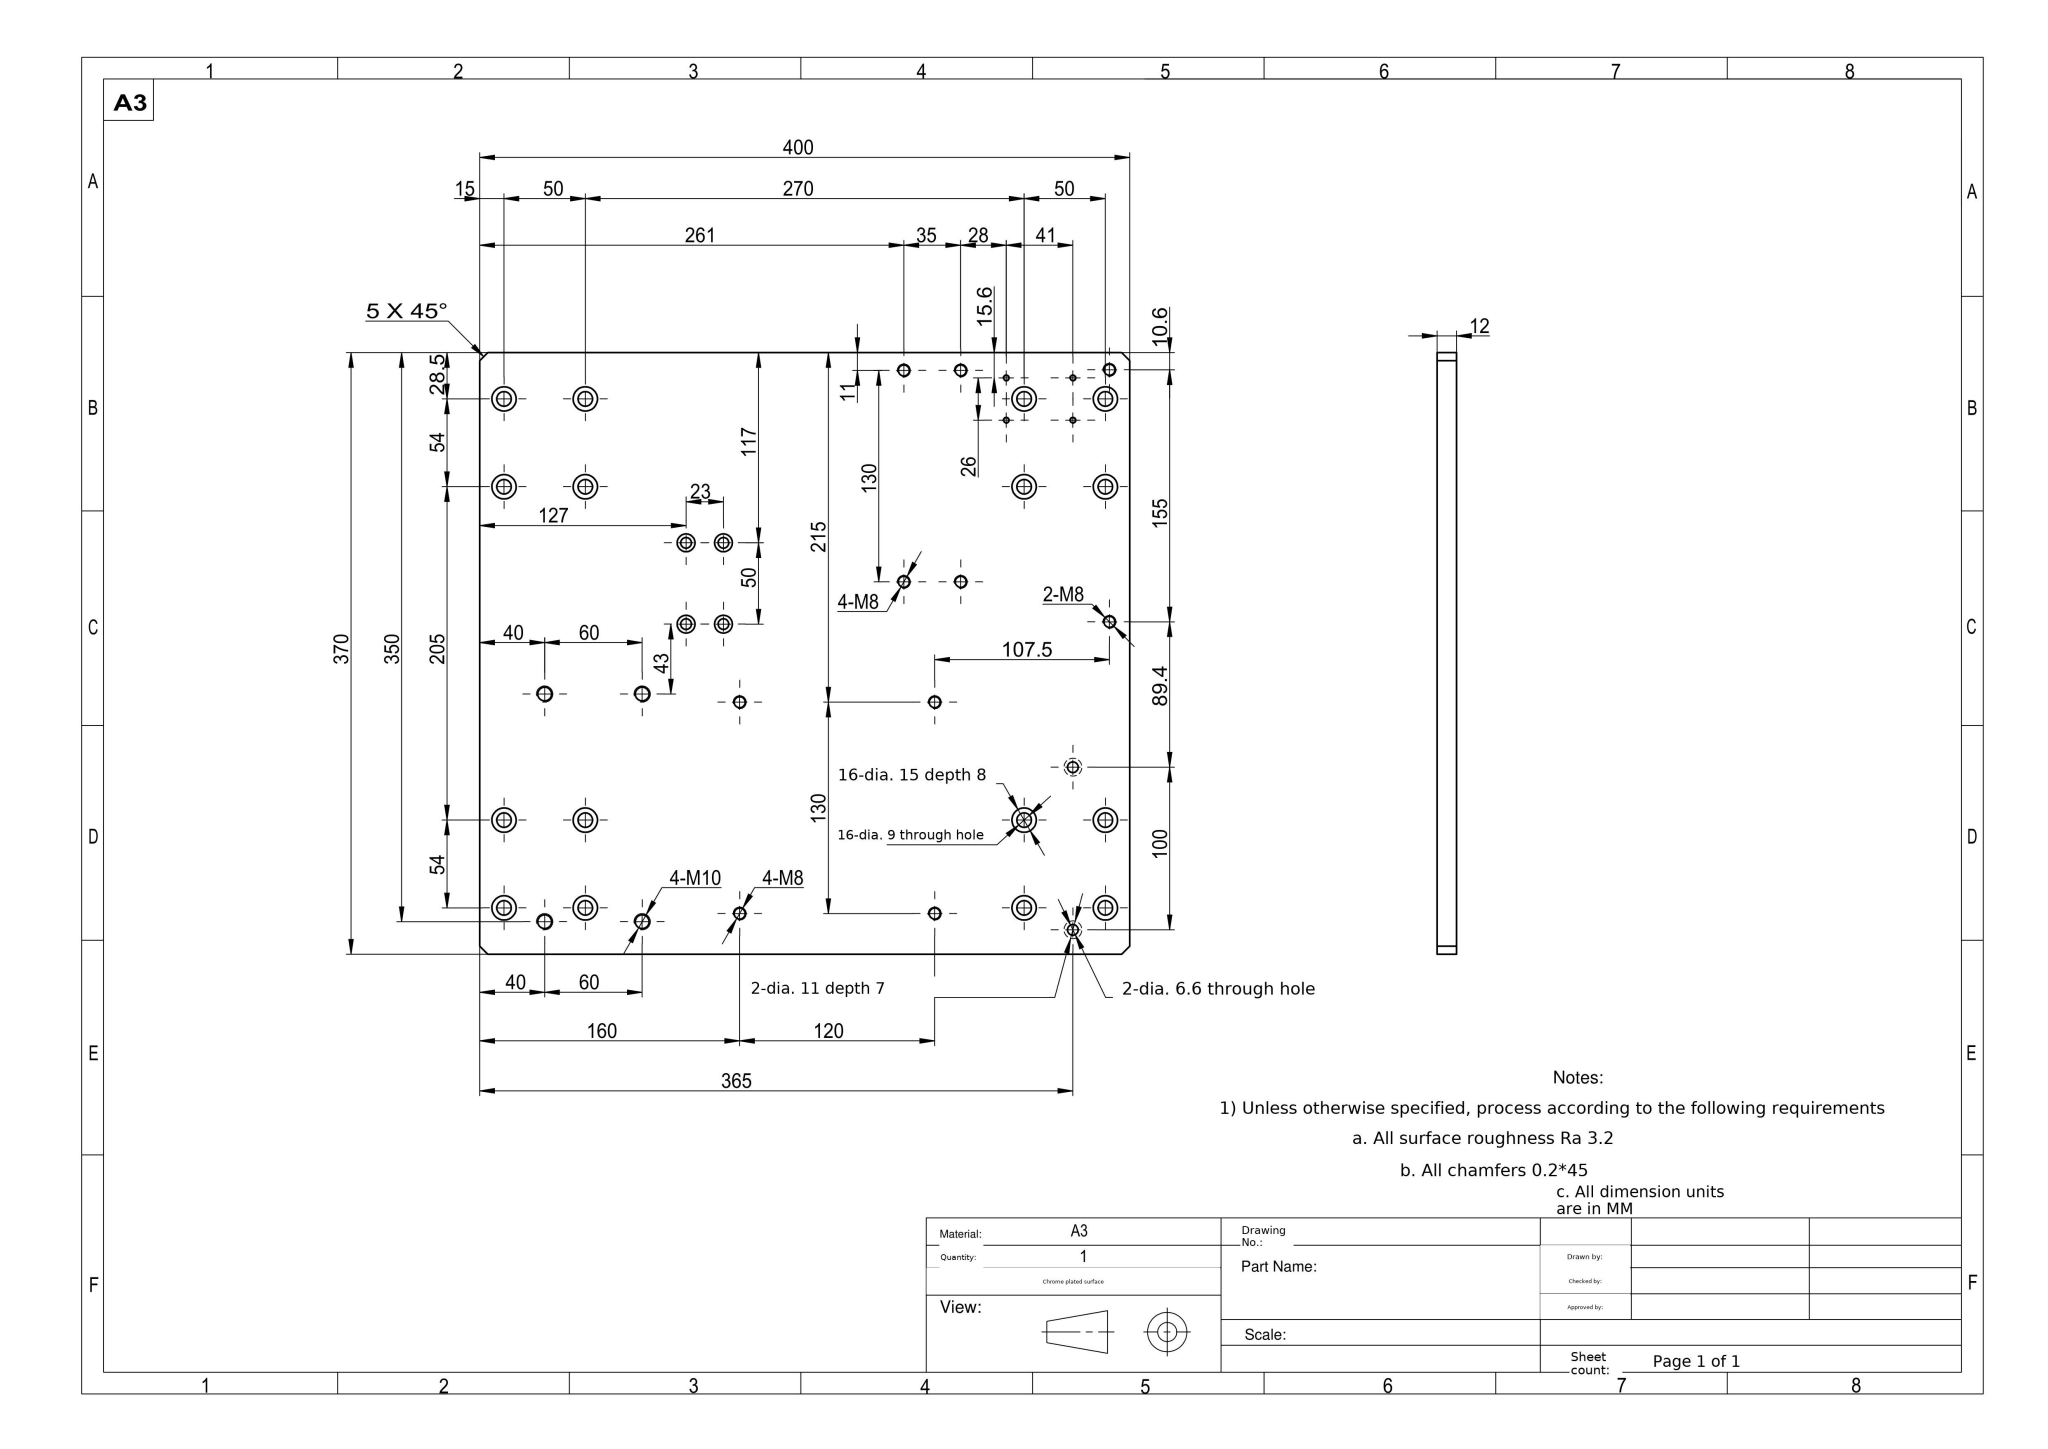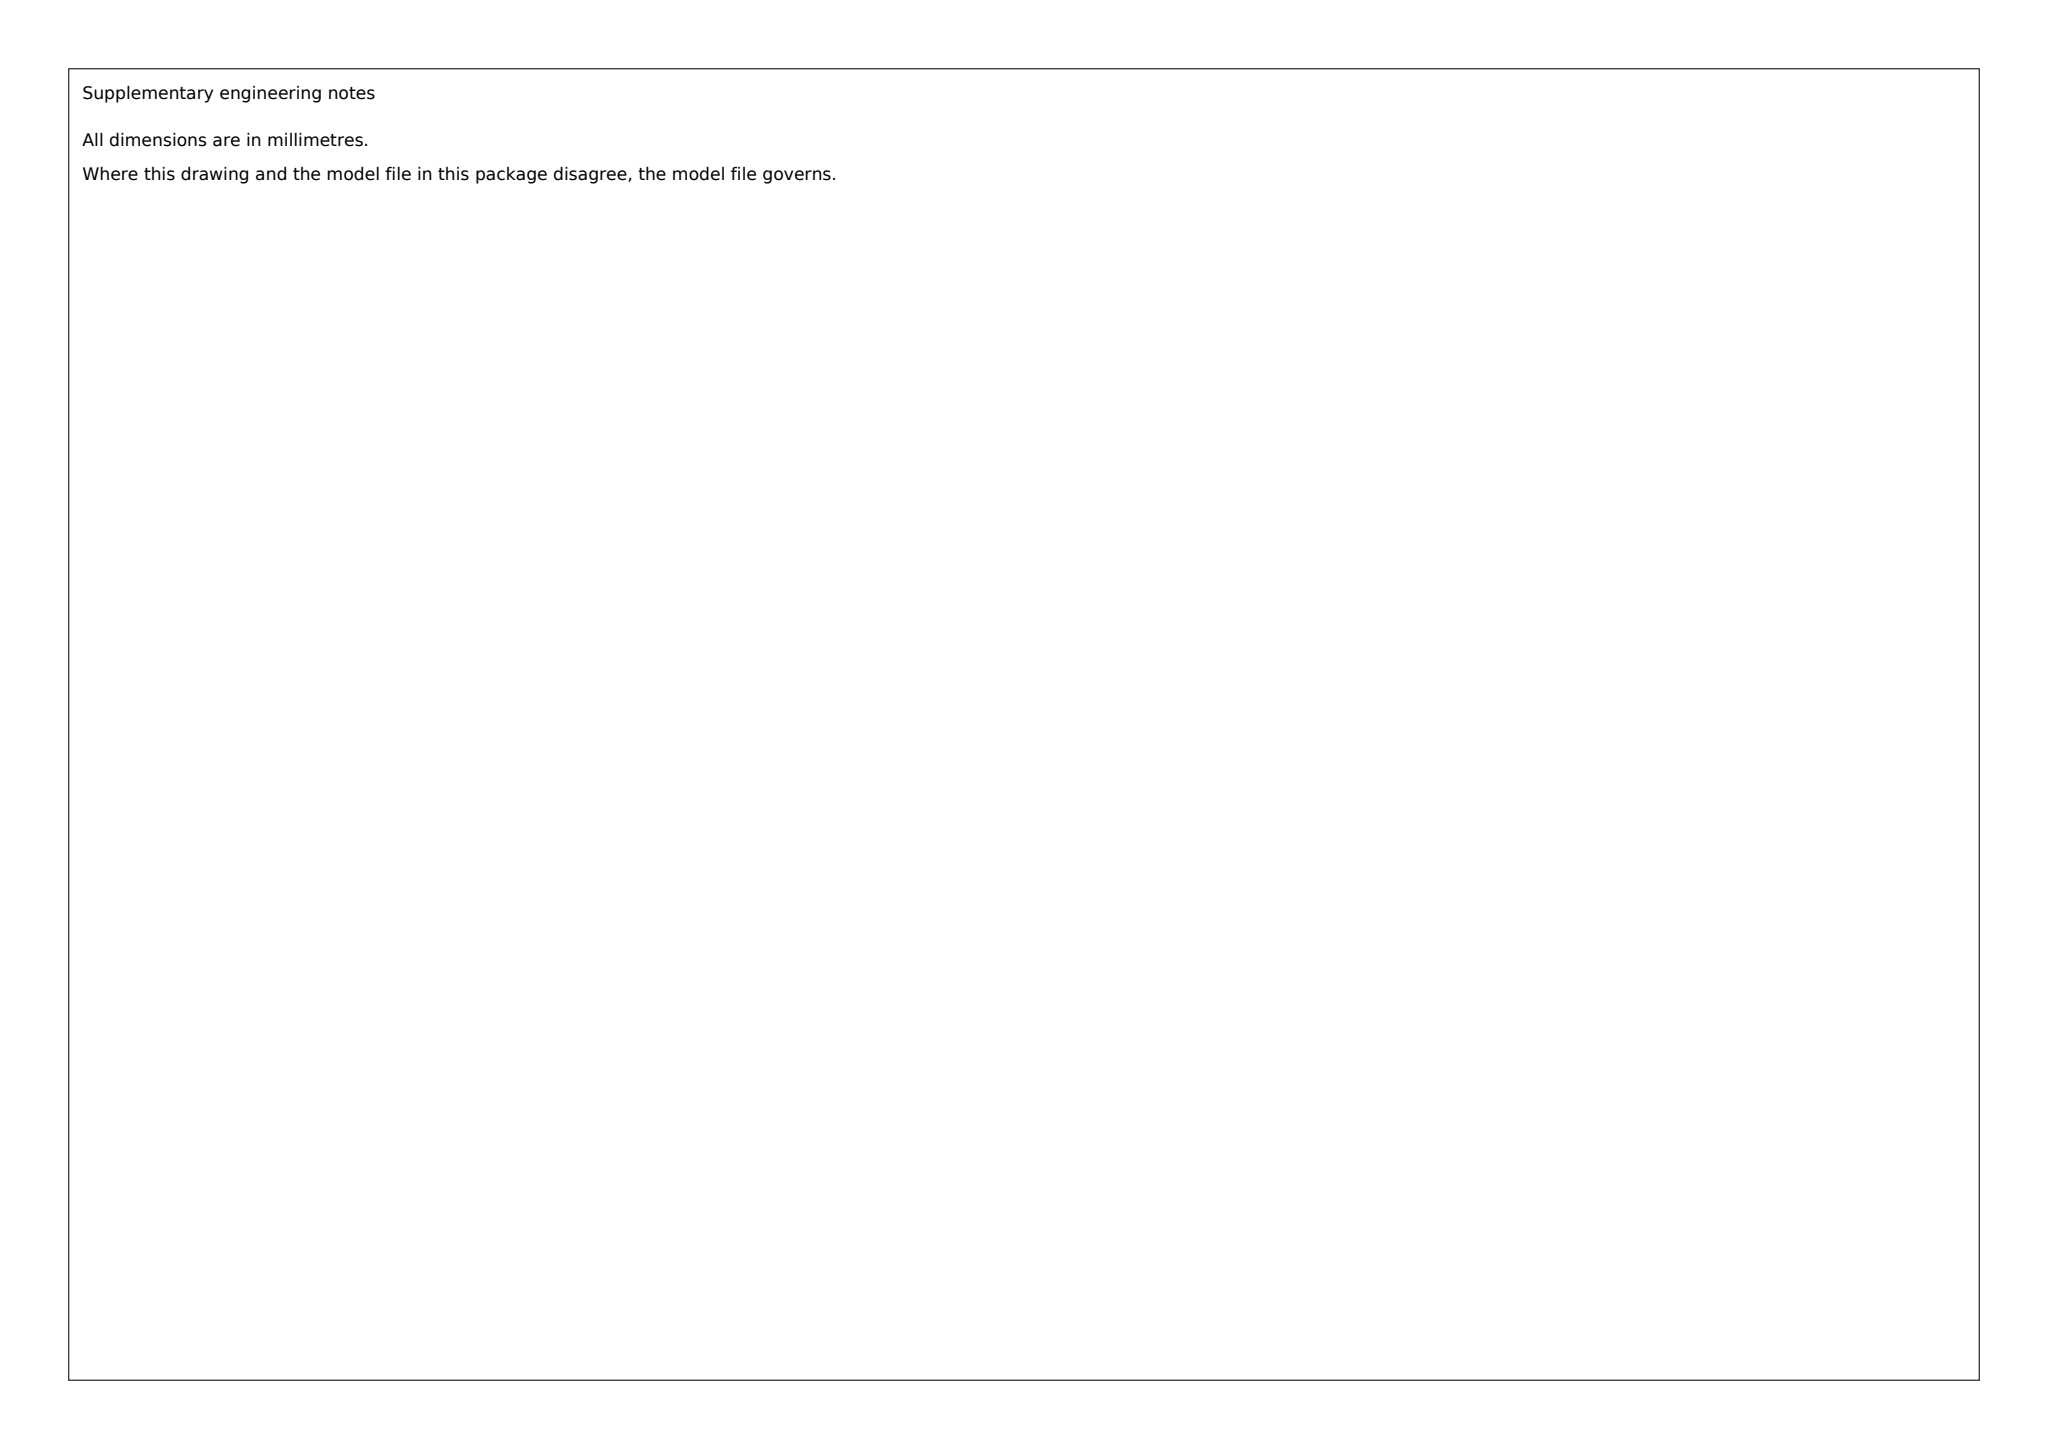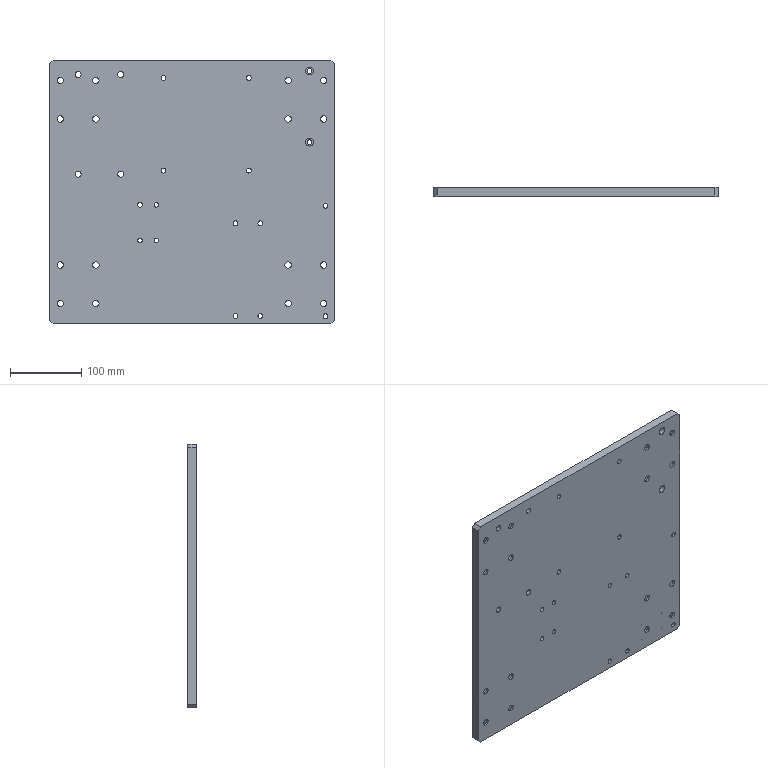Part | SolidWorks | mm | material A3 | 1 solid | 164 faces | box 400 x 12 x 370 mm | volume 1734516 mm3 | cylinder 124 | plane 32 | cone 8 | commonest cylinder face diameters 15 x32 9 x32 6.8 x20 11 x12 6.6 x12 8.5 x8 3.3 x8
build123d program:
from build123d import *

# Parameters (mm, degrees)
SKETCH1_W                                         = 400
SKETCH1_H                                         = 370
BOSS_EXTRUDE1_DEPTH                               = 6
HOLE_SIZE_ACCORDING_TO_HEXAGON_SOCKET_D           = 9
HOLE_SIZE_ACCORDING_TO_HEXAGON_SOCKET_DEPTH       = 22.25
HOLE_SIZE_ACCORDING_TO_HEXAGON_SOCKET_CBORE_D     = 15
HOLE_SIZE_ACCORDING_TO_HEXAGON_SOCKET_CBORE_DEPTH = 9
HOLE_SIZE_ACCORDING_TO_HEXAGON_SOCKET_TIP         = 2.704
HOLE_SIZE_ACCORDING_TO_HEXAGON_SO_2_D             = 6.6
HOLE_SIZE_ACCORDING_TO_HEXAGON_SO_2_DEPTH         = 15
HOLE_SIZE_ACCORDING_TO_HEXAGON_SO_2_CBORE_D       = 11
HOLE_SIZE_ACCORDING_TO_HEXAGON_SO_2_CBORE_DEPTH   = 6.8
HOLE_SIZE_ACCORDING_TO_HEXAGON_SO_2_TIP           = 1.983
M4_TAPPED_HOLE1_D                                 = 3.3
M4_TAPPED_HOLE1_DEPTH                             = 10.1
M4_TAPPED_HOLE1_TIP                               = 0.9914
M8_TAPPED_HOLE1_D                                 = 6.8
M8_TAPPED_HOLE1_DEPTH                             = 22.25
M8_TAPPED_HOLE1_TIP                               = 2.043
M8_TAPPED_HOLE2_D                                 = 6.8
M8_TAPPED_HOLE2_DEPTH                             = 19.75
M8_TAPPED_HOLE2_TIP                               = 2.043
M8_TAPPED_HOLE3_D                                 = 6.8
M8_TAPPED_HOLE3_DEPTH                             = 22.25
M8_TAPPED_HOLE3_TIP                               = 2.043
HOLE_SIZE_ACCORDING_TO_HEXAGON_SO_3_D             = 6.6
HOLE_SIZE_ACCORDING_TO_HEXAGON_SO_3_DEPTH         = 17
HOLE_SIZE_ACCORDING_TO_HEXAGON_SO_3_CBORE_D       = 11
HOLE_SIZE_ACCORDING_TO_HEXAGON_SO_3_CBORE_DEPTH   = 6.8
HOLE_SIZE_ACCORDING_TO_HEXAGON_SO_3_TIP           = 1.983
M10_TAPPED_HOLE2_D                                = 8.5
M10_TAPPED_HOLE2_DEPTH                            = 27.5
M10_TAPPED_HOLE2_TIP                              = 2.554
CHAMFER1_SIZE                                     = 5


with BuildPart() as part:
    # Sketch1 → Boss-Extrude1 (new, symmetric)
    with BuildSketch(Plane(origin=(0, 0, 0), x_dir=(1, 0, 0), z_dir=(0, 1, 0))):
        Rectangle(SKETCH1_W, SKETCH1_H)
    extrude(amount=BOSS_EXTRUDE1_DEPTH, both=True)

    # Hole Size _ according to_ Hexagon Socket
    with Locations(Plane(origin=(0, 6, 0), x_dir=(1, 0, 0), z_dir=(0, 1, 0))):
        with Locations((-185, -102.5), (-185, -156.5), (-135, -102.5), (-135, -156.5), (-135, 156.5), (-135, 102.5), (-185, 156.5), (-185, 102.5), (185, 102.5), (185, 156.5), (135, 102.5), (135, 156.5), (135, -156.5), (135, -102.5), (185, -156.5), (185, -102.5)):
            CounterBoreHole(HOLE_SIZE_ACCORDING_TO_HEXAGON_SOCKET_D / 2, HOLE_SIZE_ACCORDING_TO_HEXAGON_SOCKET_CBORE_D / 2, HOLE_SIZE_ACCORDING_TO_HEXAGON_SOCKET_CBORE_DEPTH, depth=HOLE_SIZE_ACCORDING_TO_HEXAGON_SOCKET_DEPTH)
            with Locations((0, 0, -(HOLE_SIZE_ACCORDING_TO_HEXAGON_SOCKET_DEPTH + HOLE_SIZE_ACCORDING_TO_HEXAGON_SOCKET_TIP / 2))):  # 118° drill point
                Cone(0, HOLE_SIZE_ACCORDING_TO_HEXAGON_SOCKET_D / 2, HOLE_SIZE_ACCORDING_TO_HEXAGON_SOCKET_TIP, mode=Mode.SUBTRACT)

    # Hole Size _ according to_ Hexagon So 2
    with Locations(Plane(origin=(0, -6, 0), x_dir=(-1, 0, 0), z_dir=(0, -1, 0))):
        with Locations((-165, -170), (-165, -70)):
            CounterBoreHole(HOLE_SIZE_ACCORDING_TO_HEXAGON_SO_2_D / 2, HOLE_SIZE_ACCORDING_TO_HEXAGON_SO_2_CBORE_D / 2, HOLE_SIZE_ACCORDING_TO_HEXAGON_SO_2_CBORE_DEPTH, depth=HOLE_SIZE_ACCORDING_TO_HEXAGON_SO_2_DEPTH)
            with Locations((0, 0, -(HOLE_SIZE_ACCORDING_TO_HEXAGON_SO_2_DEPTH + HOLE_SIZE_ACCORDING_TO_HEXAGON_SO_2_TIP / 2))):  # 118° drill point
                Cone(0, HOLE_SIZE_ACCORDING_TO_HEXAGON_SO_2_D / 2, HOLE_SIZE_ACCORDING_TO_HEXAGON_SO_2_TIP, mode=Mode.SUBTRACT)

    # M4 Tapped Hole1
    with Locations(Plane(origin=(0, 6, 0), x_dir=(1, 0, 0), z_dir=(0, 1, 0))):
        with Locations((124, 169.4), (124, 143.4), (165, 143.4), (165, 169.4)):
            Hole(M4_TAPPED_HOLE1_D / 2, depth=M4_TAPPED_HOLE1_DEPTH)
            with Locations((0, 0, -(M4_TAPPED_HOLE1_DEPTH + M4_TAPPED_HOLE1_TIP / 2))):  # 118° drill point
                Cone(0, M4_TAPPED_HOLE1_D / 2, M4_TAPPED_HOLE1_TIP, mode=Mode.SUBTRACT)

    # M8 Tapped Hole1
    with Locations(Plane(origin=(0, 6, 0), x_dir=(1, 0, 0), z_dir=(0, 1, 0))):
        with Locations((187.5, 19.4), (187.5, 174.4)):
            Hole(M8_TAPPED_HOLE1_D / 2, depth=M8_TAPPED_HOLE1_DEPTH)
            with Locations((0, 0, -(M8_TAPPED_HOLE1_DEPTH + M8_TAPPED_HOLE1_TIP / 2))):  # 118° drill point
                Cone(0, M8_TAPPED_HOLE1_D / 2, M8_TAPPED_HOLE1_TIP, mode=Mode.SUBTRACT)

    # M8 Tapped Hole2
    with Locations(Plane(origin=(0, 6, 0), x_dir=(1, 0, 0), z_dir=(0, 1, 0))):
        with Locations((61, 44), (61, 174), (96, 174), (96, 44)):
            Hole(M8_TAPPED_HOLE2_D / 2, depth=M8_TAPPED_HOLE2_DEPTH)
            with Locations((0, 0, -(M8_TAPPED_HOLE2_DEPTH + M8_TAPPED_HOLE2_TIP / 2))):  # 118° drill point
                Cone(0, M8_TAPPED_HOLE2_D / 2, M8_TAPPED_HOLE2_TIP, mode=Mode.SUBTRACT)

    # M8 Tapped Hole3
    with Locations(Plane(origin=(0, 6, 0), x_dir=(1, 0, 0), z_dir=(0, 1, 0))):
        with Locations((-40, -160), (80, -160), (80, -30), (-40, -30)):
            Hole(M8_TAPPED_HOLE3_D / 2, depth=M8_TAPPED_HOLE3_DEPTH)
            with Locations((0, 0, -(M8_TAPPED_HOLE3_DEPTH + M8_TAPPED_HOLE3_TIP / 2))):  # 118° drill point
                Cone(0, M8_TAPPED_HOLE3_D / 2, M8_TAPPED_HOLE3_TIP, mode=Mode.SUBTRACT)

    # Hole Size _ according to_ Hexagon So 3
    with Locations(Plane(origin=(0, 6, 0), x_dir=(1, 0, 0), z_dir=(0, 1, 0))):
        with Locations((-73, 68), (-50, 68), (-73, 18), (-50, 18)):
            CounterBoreHole(HOLE_SIZE_ACCORDING_TO_HEXAGON_SO_3_D / 2, HOLE_SIZE_ACCORDING_TO_HEXAGON_SO_3_CBORE_D / 2, HOLE_SIZE_ACCORDING_TO_HEXAGON_SO_3_CBORE_DEPTH, depth=HOLE_SIZE_ACCORDING_TO_HEXAGON_SO_3_DEPTH)
            with Locations((0, 0, -(HOLE_SIZE_ACCORDING_TO_HEXAGON_SO_3_DEPTH + HOLE_SIZE_ACCORDING_TO_HEXAGON_SO_3_TIP / 2))):  # 118° drill point
                Cone(0, HOLE_SIZE_ACCORDING_TO_HEXAGON_SO_3_D / 2, HOLE_SIZE_ACCORDING_TO_HEXAGON_SO_3_TIP, mode=Mode.SUBTRACT)

    # M10 Tapped Hole2
    with Locations(Plane(origin=(0, 6, 0), x_dir=(1, 0, 0), z_dir=(0, 1, 0))):
        with Locations((-100, -165), (-160, -165), (-100, -25), (-160, -25)):
            Hole(M10_TAPPED_HOLE2_D / 2, depth=M10_TAPPED_HOLE2_DEPTH)
            with Locations((0, 0, -(M10_TAPPED_HOLE2_DEPTH + M10_TAPPED_HOLE2_TIP / 2))):  # 118° drill point
                Cone(0, M10_TAPPED_HOLE2_D / 2, M10_TAPPED_HOLE2_TIP, mode=Mode.SUBTRACT)

    # Chamfer1
    chamfer1_edges = [part.edges().sort_by_distance(p)[0] for p in [
        (200, 0, 185),
        (-200, 0, 185),
        (-200, 0, -185),
        (200, 0, -185),
    ]]
    chamfer(chamfer1_edges, length=CHAMFER1_SIZE)


solid = part.part